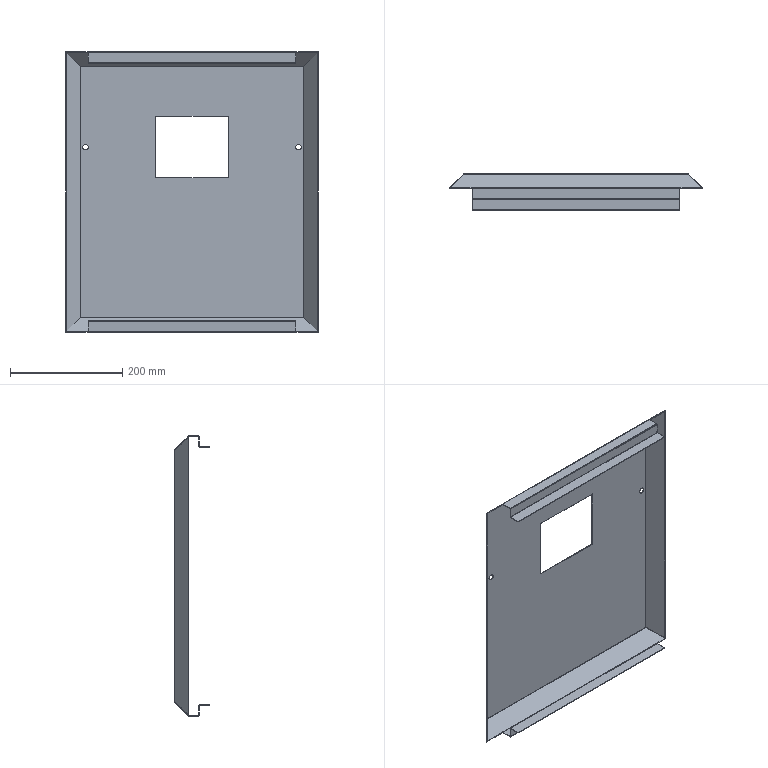Component | SolidWorks | WeldmentDrawing-1_Top-1 | 1 solid | 116 faces | volume 323440 mm3 | plane 84 | cylinder 24 | spline 8 | commonest cylinder face diameters 0.2 x10 2.6 x10 10 x4